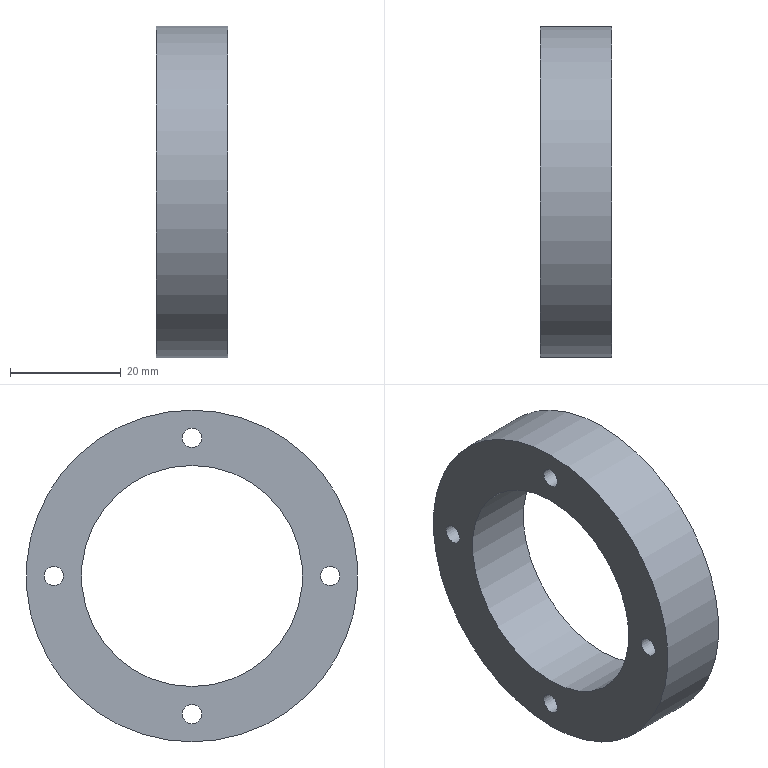Component | NX | SUPPORT_RING | 1 solid | 16 faces | volume 19323 mm3 | cylinder 10 | plane 6 | commonest cylinder face diameters 3.5 x4 6 x4 60 x1 40 x1